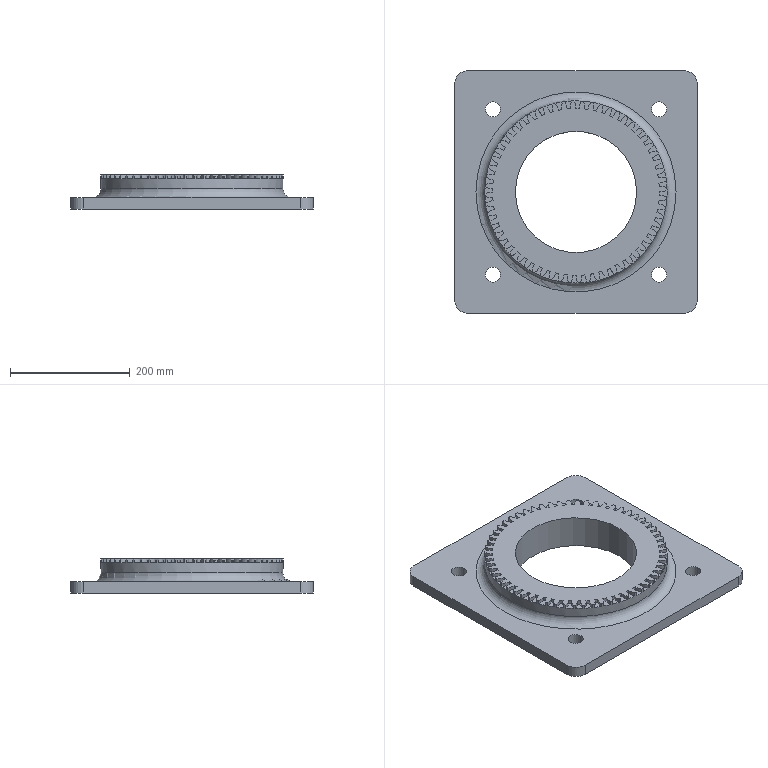Component | NX | BASE_PAD | 1 solid | 258 faces | volume 4024832 mm3 | other 120 | cylinder 70 | plane 67 | torus 1 | commonest cylinder face diameters 279.4 x60 25.4 x4 44 x4 304.8 x1 203 x1